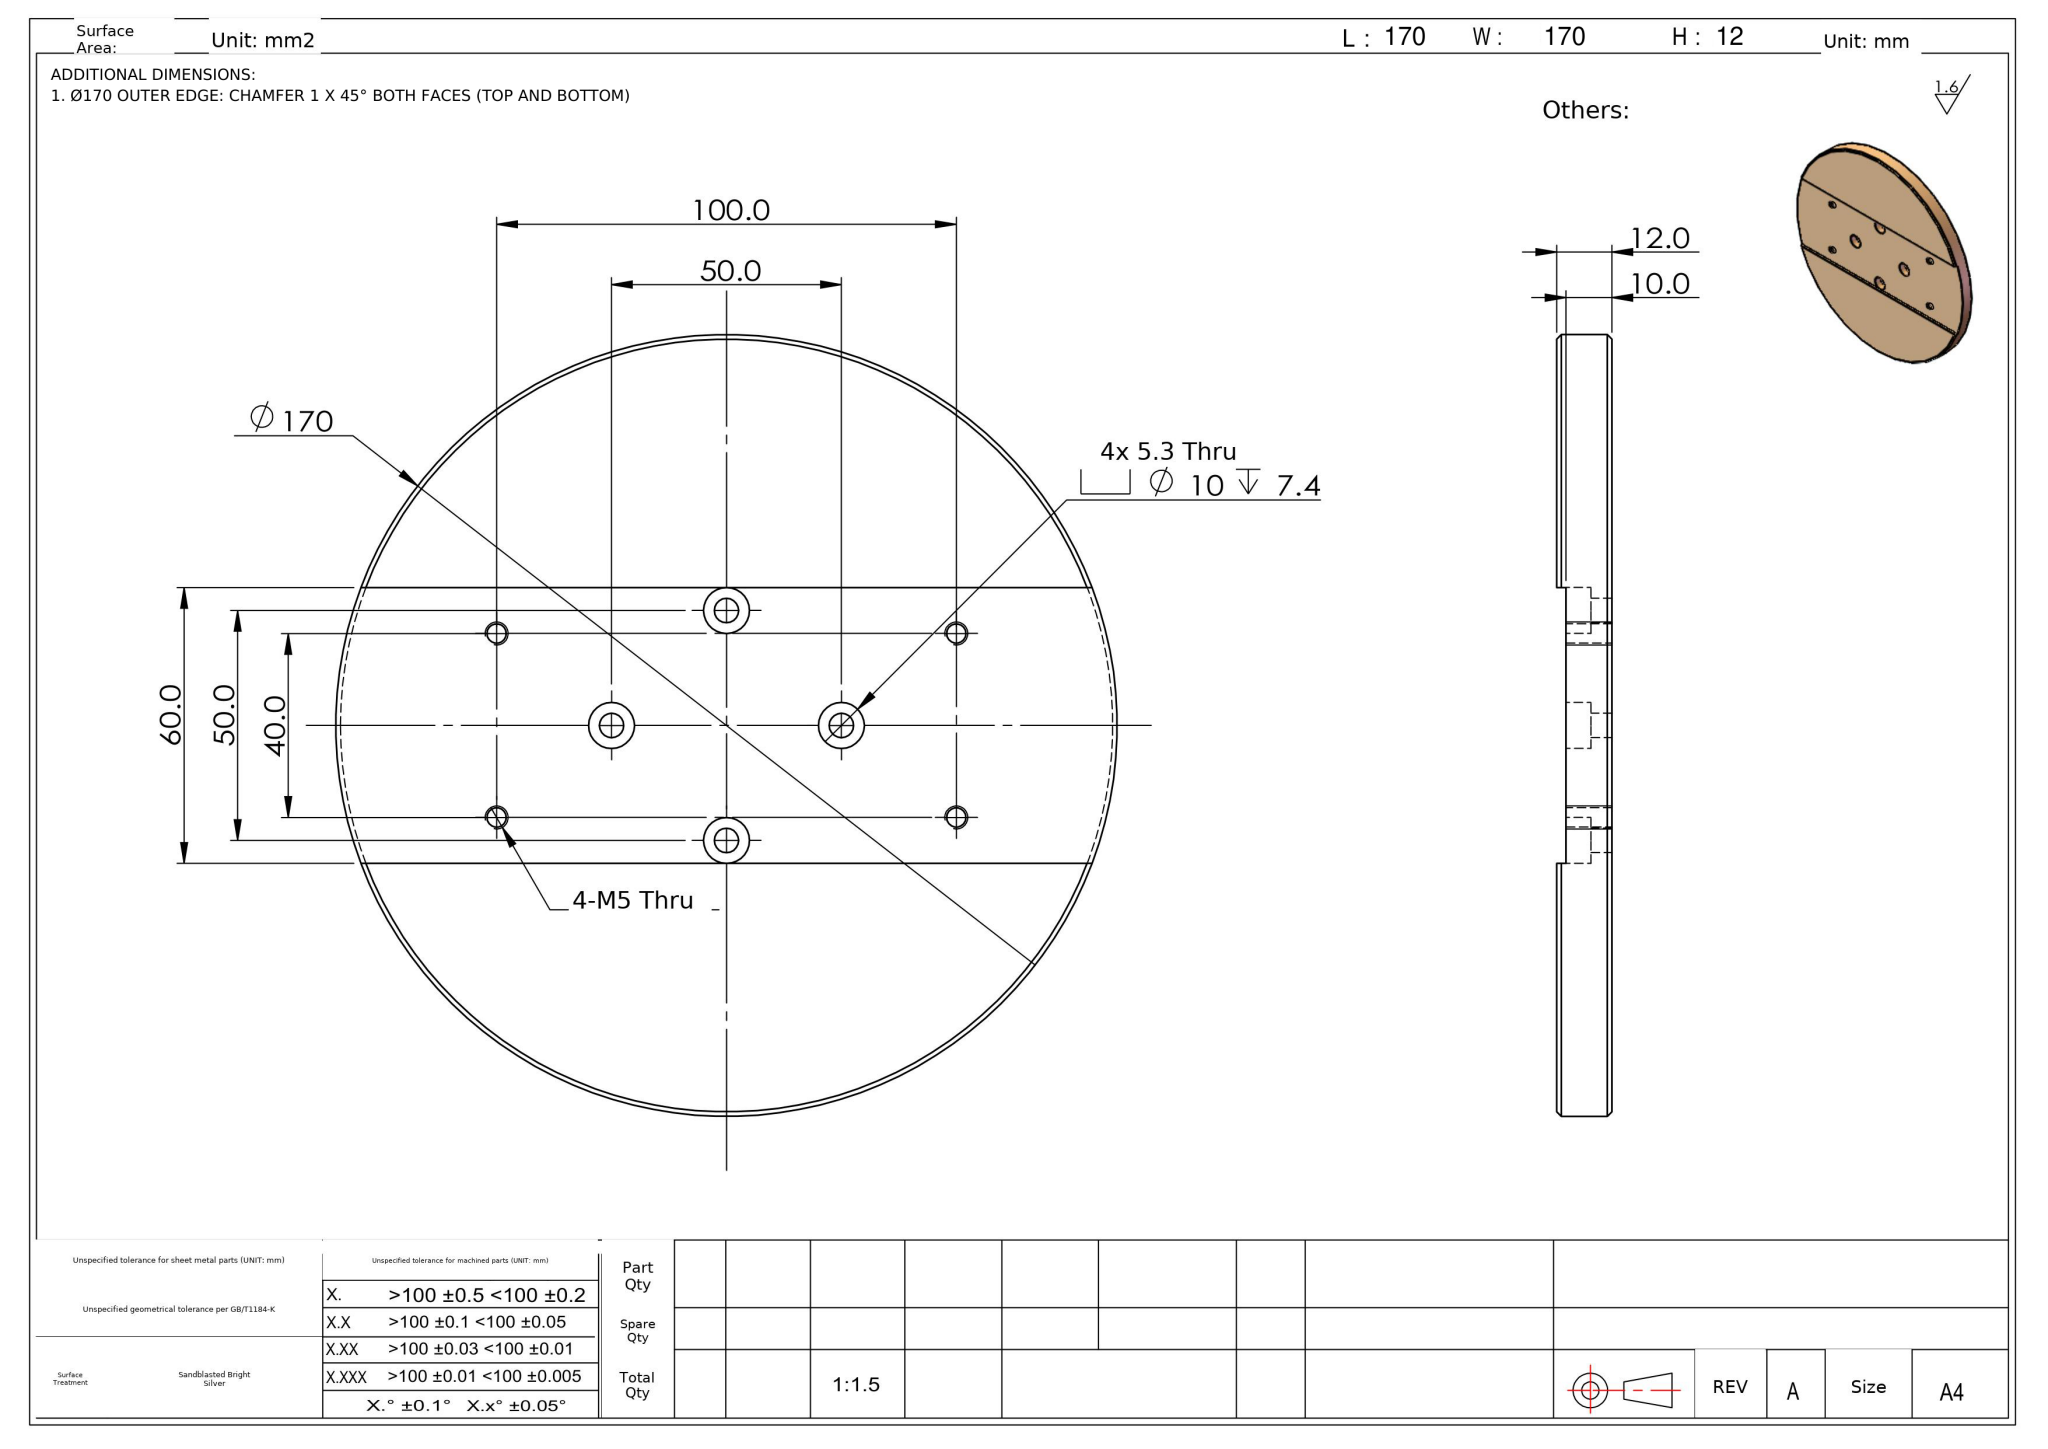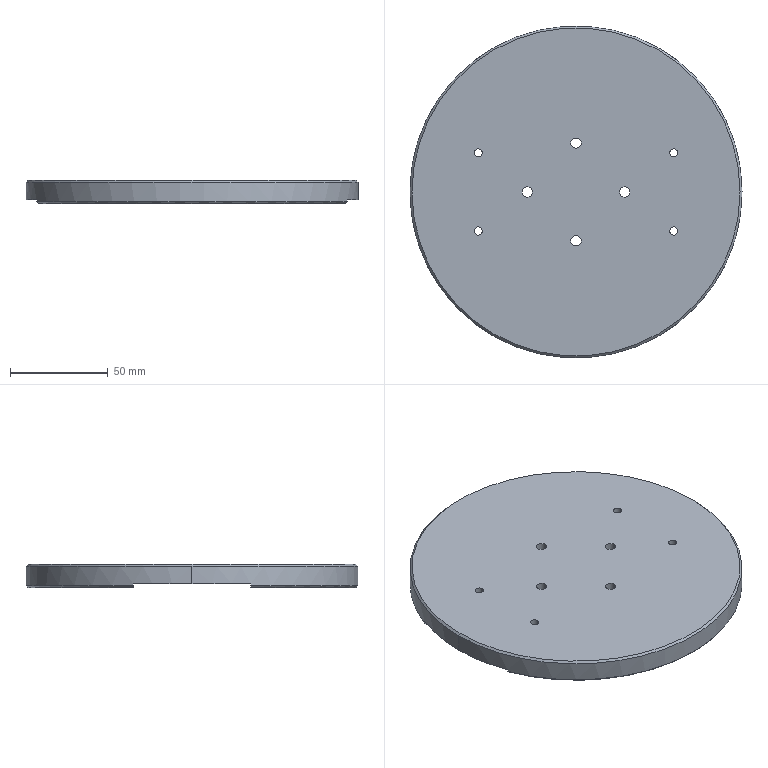Part | NX | mm | 1 solid | 40 faces | box 170 x 170 x 12 mm | volume 249281 mm3 | cylinder 26 | plane 10 | cone 4 | commonest cylinder face diameters 4.2 x8 10 x8 5.3 x8 170 x2